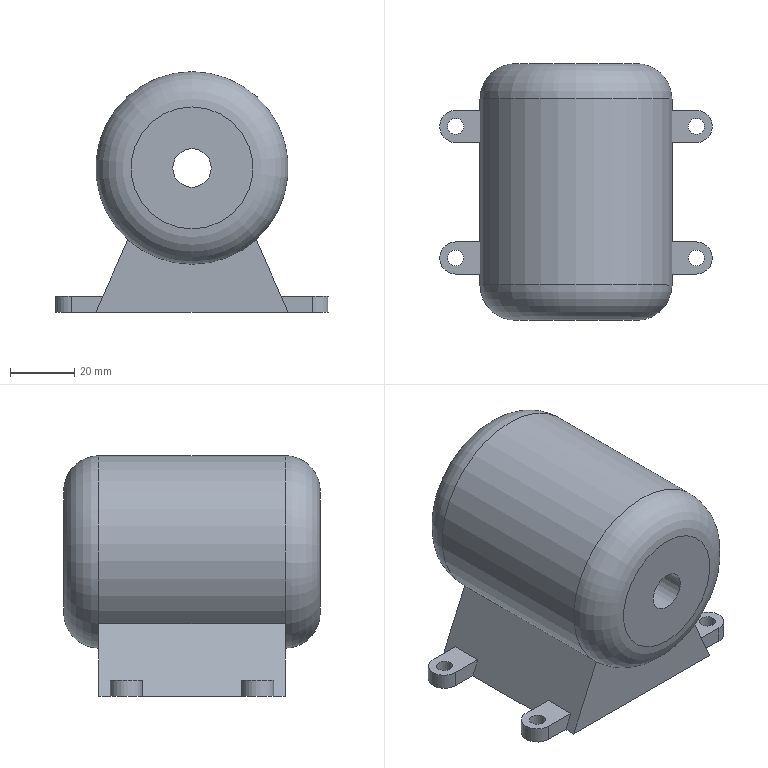Component | NX | MOTOR | 1 solid | 35 faces | volume 256139 mm3 | plane 21 | cylinder 12 | torus 2 | commonest cylinder face diameters 10 x4 5 x4 12 x2 60 x1 18 x1